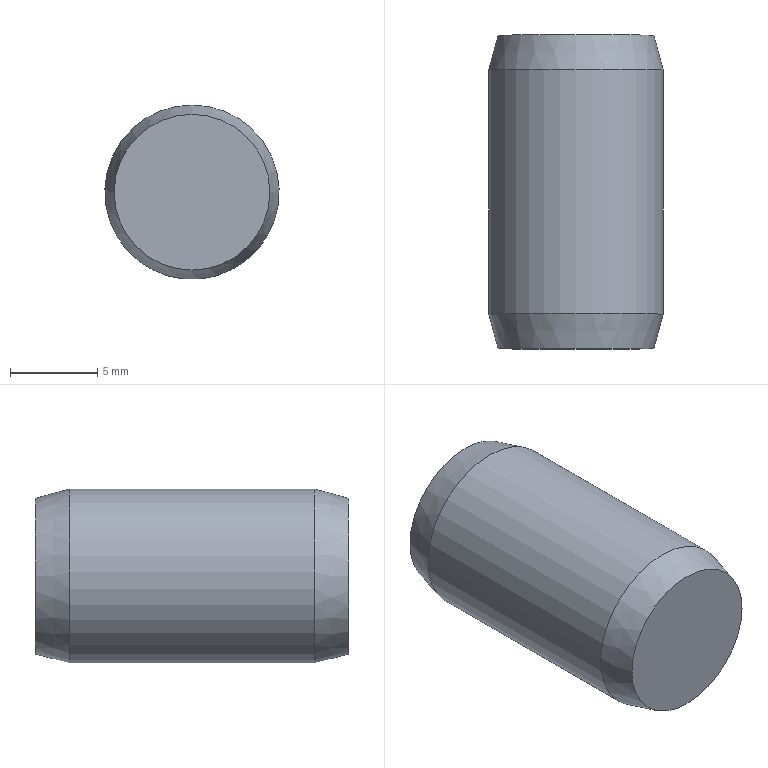Component | NX | GB-T119_1-2000_10X18_2 | 1 solid | 5 faces | box 10 x 18 x 10 mm | volume 1381 mm3 | plane 2 | cone 2 | cylinder 1 | commonest cylinder face diameters 10 x1
STEP:
#1=CARTESIAN_POINT('',(0.,0.,0.));
#2=DIRECTION('',(0.,0.,1.));
#3=DIRECTION('',(1.,0.,0.));
#4=AXIS2_PLACEMENT_3D('',#1,#2,#3);
#5=CARTESIAN_POINT('',(-69.401,-35.005,111.671));
#6=VERTEX_POINT('',#5);
#7=CARTESIAN_POINT('',(-69.401,-35.005,107.207));
#8=DIRECTION('',(0.,-1.,0.));
#9=DIRECTION('',(0.,0.,1.));
#10=AXIS2_PLACEMENT_3D('',#7,#8,#9);
#11=CIRCLE('',#10,4.464);
#12=CARTESIAN_POINT('',(-69.401,-35.005,107.207));
#13=DIRECTION('',(0.,-1.,0.));
#14=DIRECTION('',(0.,0.,1.));
#15=AXIS2_PLACEMENT_3D('',#12,#13,#14);
#16=PLANE('',#15);
#17=CARTESIAN_POINT('',(0.,0.));
#18=DIRECTION('',(1.,0.));
#19=AXIS2_PLACEMENT_2D('',#17,#18);
#20=CIRCLE('',#19,4.464);
#21=(GEOMETRIC_REPRESENTATION_CONTEXT(2)PARAMETRIC_REPRESENTATION_CONTEXT()REPRESENTATION_CONTEXT('',''));
#22=DEFINITIONAL_REPRESENTATION('',(#20),#21);
#23=PCURVE('',#16,#22);
#24=CARTESIAN_POINT('',(-69.401,-35.005,107.207));
#25=DIRECTION('',(0.,1.,0.));
#26=DIRECTION('',(0.,0.,-1.));
#27=AXIS2_PLACEMENT_3D('',#24,#25,#26);
#28=CONICAL_SURFACE('',#27,4.464,0.2618);
#29=CARTESIAN_POINT('',(9.425,0.));
#30=DIRECTION('',(-1.,0.));
#31=VECTOR('',#30,1.);
#32=LINE('',#29,#31);
#33=(GEOMETRIC_REPRESENTATION_CONTEXT(2)PARAMETRIC_REPRESENTATION_CONTEXT()REPRESENTATION_CONTEXT('',''));
#34=DEFINITIONAL_REPRESENTATION('',(#32),#33);
#35=PCURVE('',#28,#34);
#36=SURFACE_CURVE('',#11,(#23,#35),.PCURVE_S1.);
#37=EDGE_CURVE('',#6,#6,#36,.T.);
#38=ORIENTED_EDGE('',*,*,#37,.T.);
#39=EDGE_LOOP('',(#38));
#40=FACE_BOUND('',#39,.T.);
#41=ADVANCED_FACE('',(#40),#16,.T.);
#42=CARTESIAN_POINT('',(-69.401,-33.005,112.207));
#43=VERTEX_POINT('',#42);
#44=CARTESIAN_POINT('',(-69.401,-33.005,107.207));
#45=DIRECTION('',(0.,-1.,0.));
#46=DIRECTION('',(0.,0.,1.));
#47=AXIS2_PLACEMENT_3D('',#44,#45,#46);
#48=CIRCLE('',#47,5.);
#49=CARTESIAN_POINT('',(9.425,2.));
#50=DIRECTION('',(-1.,0.));
#51=VECTOR('',#50,1.);
#52=LINE('',#49,#51);
#53=(GEOMETRIC_REPRESENTATION_CONTEXT(2)PARAMETRIC_REPRESENTATION_CONTEXT()REPRESENTATION_CONTEXT('',''));
#54=DEFINITIONAL_REPRESENTATION('',(#52),#53);
#55=PCURVE('',#28,#54);
#56=CARTESIAN_POINT('',(-69.401,-17.005,107.207));
#57=DIRECTION('',(0.,-1.,0.));
#58=DIRECTION('',(0.,0.,1.));
#59=AXIS2_PLACEMENT_3D('',#56,#57,#58);
#60=CYLINDRICAL_SURFACE('',#59,5.);
#61=CARTESIAN_POINT('',(0.,16.));
#62=DIRECTION('',(1.,0.));
#63=VECTOR('',#62,1.);
#64=LINE('',#61,#63);
#65=(GEOMETRIC_REPRESENTATION_CONTEXT(2)PARAMETRIC_REPRESENTATION_CONTEXT()REPRESENTATION_CONTEXT('',''));
#66=DEFINITIONAL_REPRESENTATION('',(#64),#65);
#67=PCURVE('',#60,#66);
#68=SURFACE_CURVE('',#48,(#55,#67),.PCURVE_S1.);
#69=EDGE_CURVE('',#43,#43,#68,.T.);
#70=ORIENTED_EDGE('',*,*,#69,.T.);
#71=CARTESIAN_POINT('',(-69.401,-35.005,111.671));
#72=CARTESIAN_POINT('',(-69.401,-33.005,112.207));
#73=B_SPLINE_CURVE_WITH_KNOTS('',1,(#71,#72),.UNSPECIFIED.,.F.,.F.,(2,2),(0.,2.071),.PIECEWISE_BEZIER_KNOTS.);
#74=CARTESIAN_POINT('',(3.142,0.));
#75=DIRECTION('',(0.,1.));
#76=VECTOR('',#75,1.);
#77=LINE('',#74,#76);
#78=(GEOMETRIC_REPRESENTATION_CONTEXT(2)PARAMETRIC_REPRESENTATION_CONTEXT()REPRESENTATION_CONTEXT('',''));
#79=DEFINITIONAL_REPRESENTATION('',(#77),#78);
#80=PCURVE('',#28,#79);
#81=CARTESIAN_POINT('',(9.425,0.));
#82=DIRECTION('',(0.,1.));
#83=VECTOR('',#82,1.);
#84=LINE('',#81,#83);
#85=(GEOMETRIC_REPRESENTATION_CONTEXT(2)PARAMETRIC_REPRESENTATION_CONTEXT()REPRESENTATION_CONTEXT('',''));
#86=DEFINITIONAL_REPRESENTATION('',(#84),#85);
#87=PCURVE('',#28,#86);
#88=SEAM_CURVE('',#73,(#80,#87),.PCURVE_S1.);
#89=EDGE_CURVE('',#6,#43,#88,.T.);
#90=ORIENTED_EDGE('',*,*,#89,.F.);
#91=ORIENTED_EDGE('',*,*,#37,.F.);
#92=ORIENTED_EDGE('',*,*,#89,.T.);
#93=EDGE_LOOP('',(#70,#90,#91,#92));
#94=FACE_BOUND('',#93,.T.);
#95=ADVANCED_FACE('',(#94),#28,.T.);
#96=CARTESIAN_POINT('',(-69.401,-19.005,112.207));
#97=VERTEX_POINT('',#96);
#98=CARTESIAN_POINT('',(-69.401,-19.005,107.207));
#99=DIRECTION('',(0.,-1.,0.));
#100=DIRECTION('',(0.,0.,1.));
#101=AXIS2_PLACEMENT_3D('',#98,#99,#100);
#102=CIRCLE('',#101,5.);
#103=CARTESIAN_POINT('',(0.,2.));
#104=DIRECTION('',(1.,0.));
#105=VECTOR('',#104,1.);
#106=LINE('',#103,#105);
#107=(GEOMETRIC_REPRESENTATION_CONTEXT(2)PARAMETRIC_REPRESENTATION_CONTEXT()REPRESENTATION_CONTEXT('',''));
#108=DEFINITIONAL_REPRESENTATION('',(#106),#107);
#109=PCURVE('',#60,#108);
#110=CARTESIAN_POINT('',(-69.401,-19.005,107.207));
#111=DIRECTION('',(0.,-1.,0.));
#112=DIRECTION('',(0.,0.,1.));
#113=AXIS2_PLACEMENT_3D('',#110,#111,#112);
#114=CONICAL_SURFACE('',#113,5.,0.2618);
#115=CARTESIAN_POINT('',(0.,0.));
#116=DIRECTION('',(1.,0.));
#117=VECTOR('',#116,1.);
#118=LINE('',#115,#117);
#119=(GEOMETRIC_REPRESENTATION_CONTEXT(2)PARAMETRIC_REPRESENTATION_CONTEXT()REPRESENTATION_CONTEXT('',''));
#120=DEFINITIONAL_REPRESENTATION('',(#118),#119);
#121=PCURVE('',#114,#120);
#122=SURFACE_CURVE('',#102,(#109,#121),.PCURVE_S1.);
#123=EDGE_CURVE('',#97,#97,#122,.T.);
#124=ORIENTED_EDGE('',*,*,#123,.T.);
#125=CARTESIAN_POINT('',(-69.401,-19.005,112.207));
#126=CARTESIAN_POINT('',(-69.401,-33.005,112.207));
#127=B_SPLINE_CURVE_WITH_KNOTS('',1,(#125,#126),.UNSPECIFIED.,.F.,.F.,(2,2),(2.,16.),.PIECEWISE_BEZIER_KNOTS.);
#128=CARTESIAN_POINT('',(6.283,0.));
#129=DIRECTION('',(0.,1.));
#130=VECTOR('',#129,1.);
#131=LINE('',#128,#130);
#132=(GEOMETRIC_REPRESENTATION_CONTEXT(2)PARAMETRIC_REPRESENTATION_CONTEXT()REPRESENTATION_CONTEXT('',''));
#133=DEFINITIONAL_REPRESENTATION('',(#131),#132);
#134=PCURVE('',#60,#133);
#135=CARTESIAN_POINT('',(0.,0.));
#136=DIRECTION('',(0.,1.));
#137=VECTOR('',#136,1.);
#138=LINE('',#135,#137);
#139=(GEOMETRIC_REPRESENTATION_CONTEXT(2)PARAMETRIC_REPRESENTATION_CONTEXT()REPRESENTATION_CONTEXT('',''));
#140=DEFINITIONAL_REPRESENTATION('',(#138),#139);
#141=PCURVE('',#60,#140);
#142=SEAM_CURVE('',#127,(#134,#141),.PCURVE_S1.);
#143=EDGE_CURVE('',#97,#43,#142,.T.);
#144=ORIENTED_EDGE('',*,*,#143,.T.);
#145=ORIENTED_EDGE('',*,*,#69,.F.);
#146=ORIENTED_EDGE('',*,*,#143,.F.);
#147=EDGE_LOOP('',(#124,#144,#145,#146));
#148=FACE_BOUND('',#147,.T.);
#149=ADVANCED_FACE('',(#148),#60,.T.);
#150=CARTESIAN_POINT('',(-69.401,-17.005,111.671));
#151=VERTEX_POINT('',#150);
#152=CARTESIAN_POINT('',(-69.401,-17.005,107.207));
#153=DIRECTION('',(0.,-1.,0.));
#154=DIRECTION('',(0.,0.,1.));
#155=AXIS2_PLACEMENT_3D('',#152,#153,#154);
#156=CIRCLE('',#155,4.464);
#157=CARTESIAN_POINT('',(0.,-2.));
#158=DIRECTION('',(1.,0.));
#159=VECTOR('',#158,1.);
#160=LINE('',#157,#159);
#161=(GEOMETRIC_REPRESENTATION_CONTEXT(2)PARAMETRIC_REPRESENTATION_CONTEXT()REPRESENTATION_CONTEXT('',''));
#162=DEFINITIONAL_REPRESENTATION('',(#160),#161);
#163=PCURVE('',#114,#162);
#164=CARTESIAN_POINT('',(-69.401,-17.005,102.743));
#165=DIRECTION('',(0.,1.,0.));
#166=DIRECTION('',(0.,0.,-1.));
#167=AXIS2_PLACEMENT_3D('',#164,#165,#166);
#168=PLANE('',#167);
#169=CARTESIAN_POINT('',(-8.928,0.));
#170=CARTESIAN_POINT('',(-8.928,7.732));
#171=CARTESIAN_POINT('',(-2.232,3.866));
#172=CARTESIAN_POINT('',(4.464,0.));
#173=CARTESIAN_POINT('',(-2.232,-3.866));
#174=CARTESIAN_POINT('',(-8.928,-7.732));
#175=CARTESIAN_POINT('',(-8.928,0.));
#176=(BOUNDED_CURVE()B_SPLINE_CURVE(2,(#169,#170,#171,#172,#173,#174,#175),.UNSPECIFIED.,.T.,.F.)B_SPLINE_CURVE_WITH_KNOTS((1,2,2,2,2,1),(-2.094,0.,2.094,4.189,6.283,8.378),.UNSPECIFIED.)CURVE()GEOMETRIC_REPRESENTATION_ITEM()RATIONAL_B_SPLINE_CURVE((1.,0.5,1.,0.5,1.,0.5,1.))REPRESENTATION_ITEM(''));
#177=(GEOMETRIC_REPRESENTATION_CONTEXT(2)PARAMETRIC_REPRESENTATION_CONTEXT()REPRESENTATION_CONTEXT('',''));
#178=DEFINITIONAL_REPRESENTATION('',(#176),#177);
#179=PCURVE('',#168,#178);
#180=SURFACE_CURVE('',#156,(#163,#179),.PCURVE_S1.);
#181=EDGE_CURVE('',#151,#151,#180,.T.);
#182=ORIENTED_EDGE('',*,*,#181,.T.);
#183=CARTESIAN_POINT('',(-69.401,-17.005,111.671));
#184=CARTESIAN_POINT('',(-69.401,-19.005,112.207));
#185=B_SPLINE_CURVE_WITH_KNOTS('',1,(#183,#184),.UNSPECIFIED.,.F.,.F.,(2,2),(-2.071,0.),.PIECEWISE_BEZIER_KNOTS.);
#186=CARTESIAN_POINT('',(6.283,0.));
#187=DIRECTION('',(0.,1.));
#188=VECTOR('',#187,1.);
#189=LINE('',#186,#188);
#190=(GEOMETRIC_REPRESENTATION_CONTEXT(2)PARAMETRIC_REPRESENTATION_CONTEXT()REPRESENTATION_CONTEXT('',''));
#191=DEFINITIONAL_REPRESENTATION('',(#189),#190);
#192=PCURVE('',#114,#191);
#193=CARTESIAN_POINT('',(0.,0.));
#194=DIRECTION('',(0.,1.));
#195=VECTOR('',#194,1.);
#196=LINE('',#193,#195);
#197=(GEOMETRIC_REPRESENTATION_CONTEXT(2)PARAMETRIC_REPRESENTATION_CONTEXT()REPRESENTATION_CONTEXT('',''));
#198=DEFINITIONAL_REPRESENTATION('',(#196),#197);
#199=PCURVE('',#114,#198);
#200=SEAM_CURVE('',#185,(#192,#199),.PCURVE_S1.);
#201=EDGE_CURVE('',#151,#97,#200,.T.);
#202=ORIENTED_EDGE('',*,*,#201,.T.);
#203=ORIENTED_EDGE('',*,*,#123,.F.);
#204=ORIENTED_EDGE('',*,*,#201,.F.);
#205=EDGE_LOOP('',(#182,#202,#203,#204));
#206=FACE_BOUND('',#205,.T.);
#207=ADVANCED_FACE('',(#206),#114,.T.);
#208=ORIENTED_EDGE('',*,*,#181,.F.);
#209=EDGE_LOOP('',(#208));
#210=FACE_BOUND('',#209,.T.);
#211=ADVANCED_FACE('',(#210),#168,.T.);
#212=CLOSED_SHELL('',(#41,#95,#149,#207,#211));
#213=MANIFOLD_SOLID_BREP('',#212);
#214=(LENGTH_UNIT()NAMED_UNIT(*)SI_UNIT(.MILLI.,.METRE.));
#215=UNCERTAINTY_MEASURE_WITH_UNIT(LENGTH_MEASURE(0.00001),#214,'','');
#216=(NAMED_UNIT(*)PLANE_ANGLE_UNIT()SI_UNIT($,.RADIAN.));
#217=(NAMED_UNIT(*)SI_UNIT($,.STERADIAN.)SOLID_ANGLE_UNIT());
#218=(GEOMETRIC_REPRESENTATION_CONTEXT(3)GLOBAL_UNCERTAINTY_ASSIGNED_CONTEXT((#215))GLOBAL_UNIT_ASSIGNED_CONTEXT((#214,#216,#217))REPRESENTATION_CONTEXT('',''));
#219=ADVANCED_BREP_SHAPE_REPRESENTATION('',(#4,#213),#218);